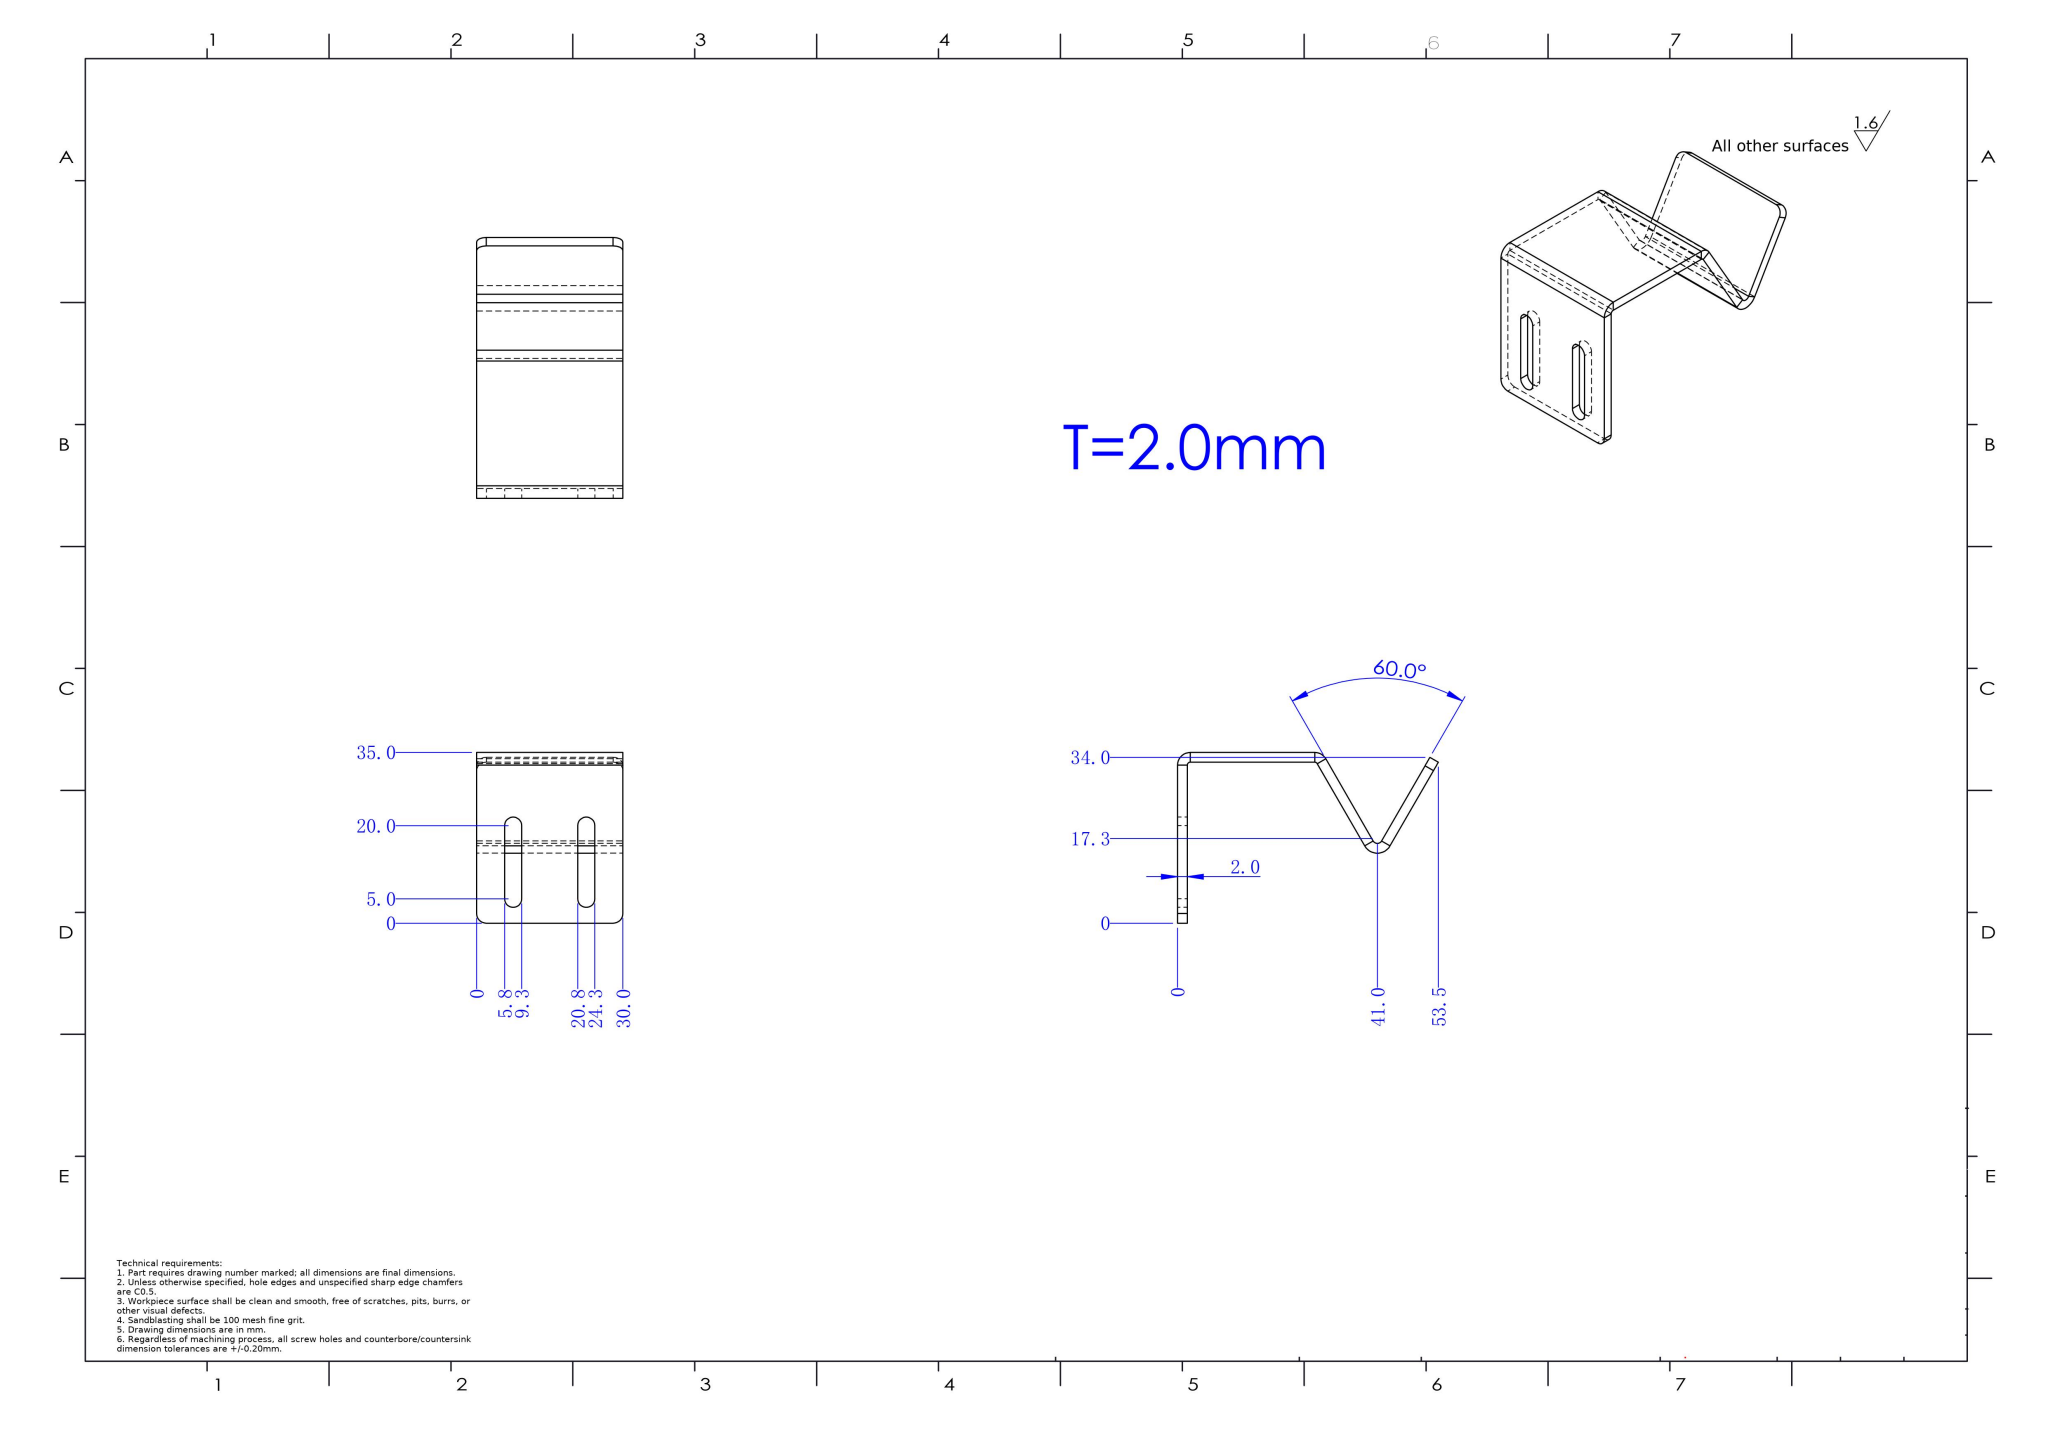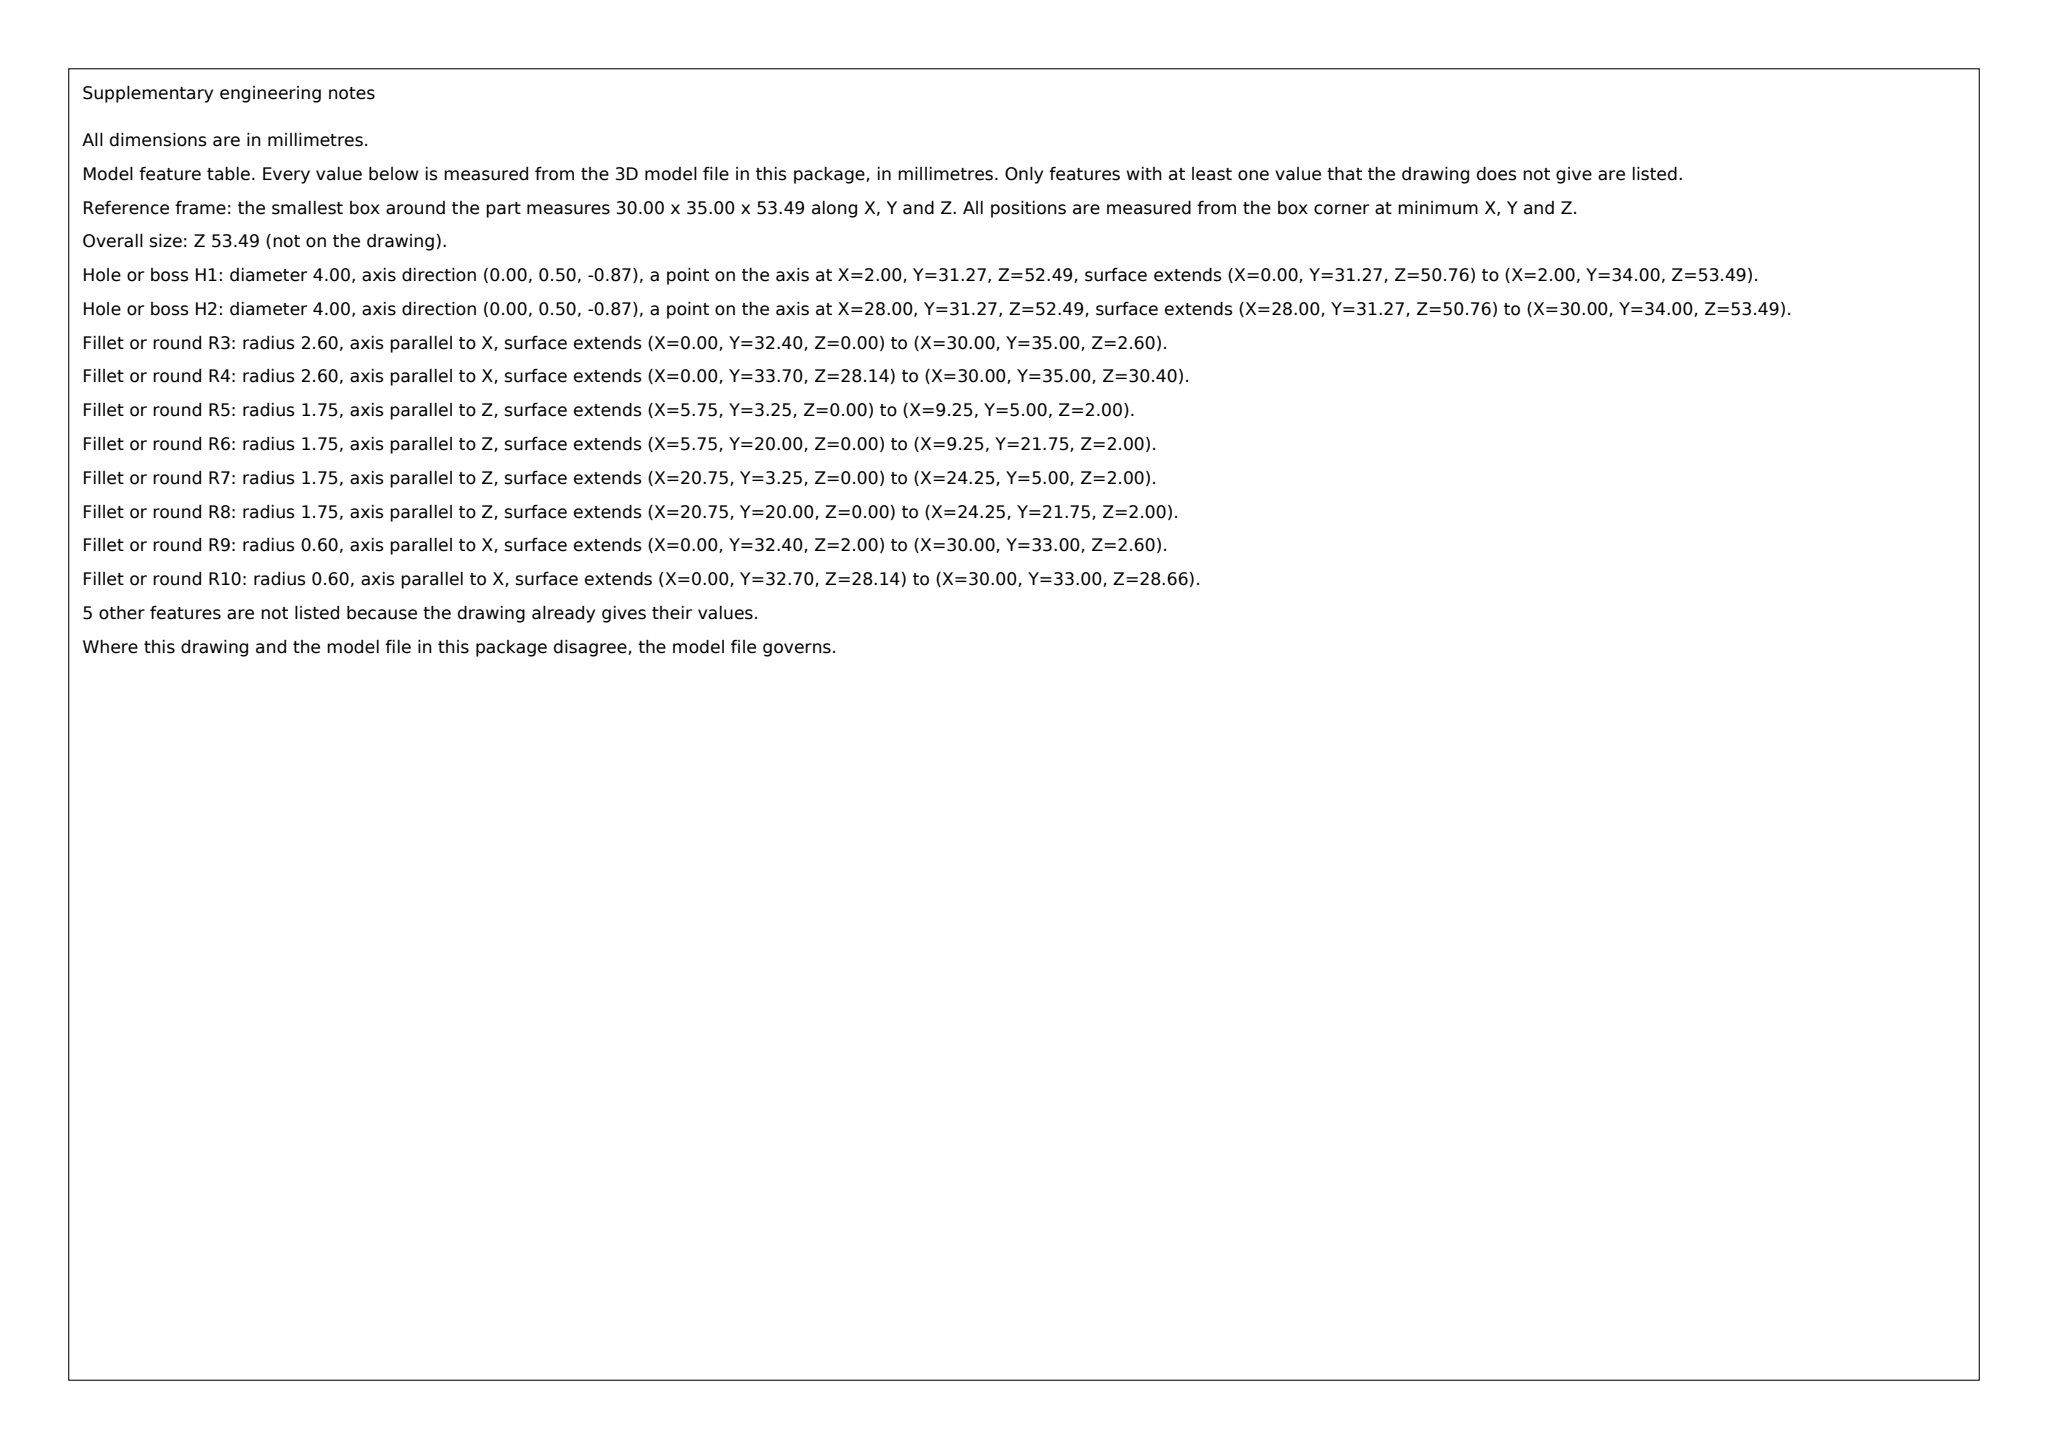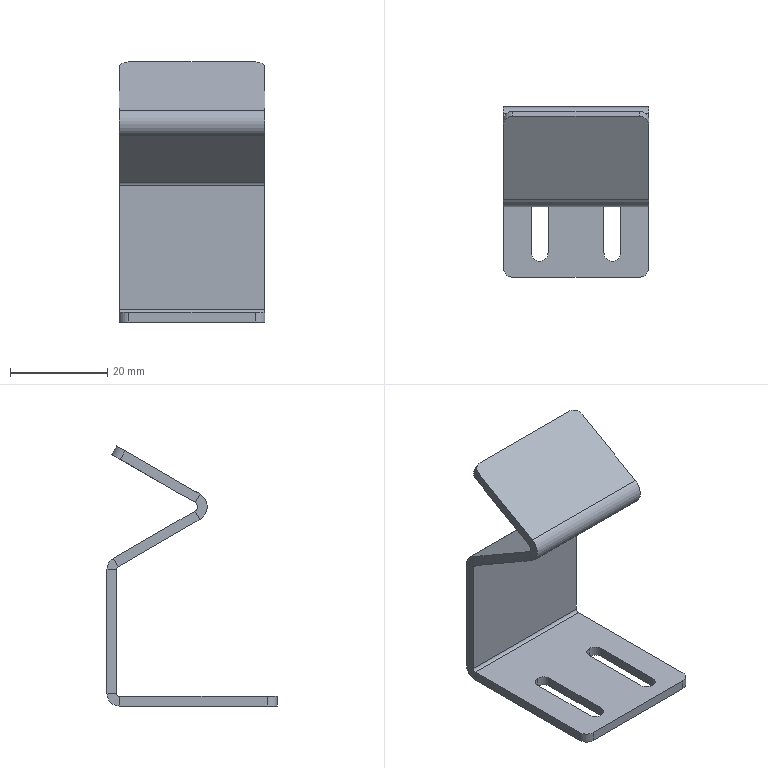Part | SolidWorks | mm | 1 solid | 44 faces | box 30 x 35 x 53.49 mm | volume 6080 mm3 | plane 28 | cylinder 16 | commonest cylinder face diameters 3.5 x6 4 x4 5.2 x2 1.2 x2 6 x1 2 x1